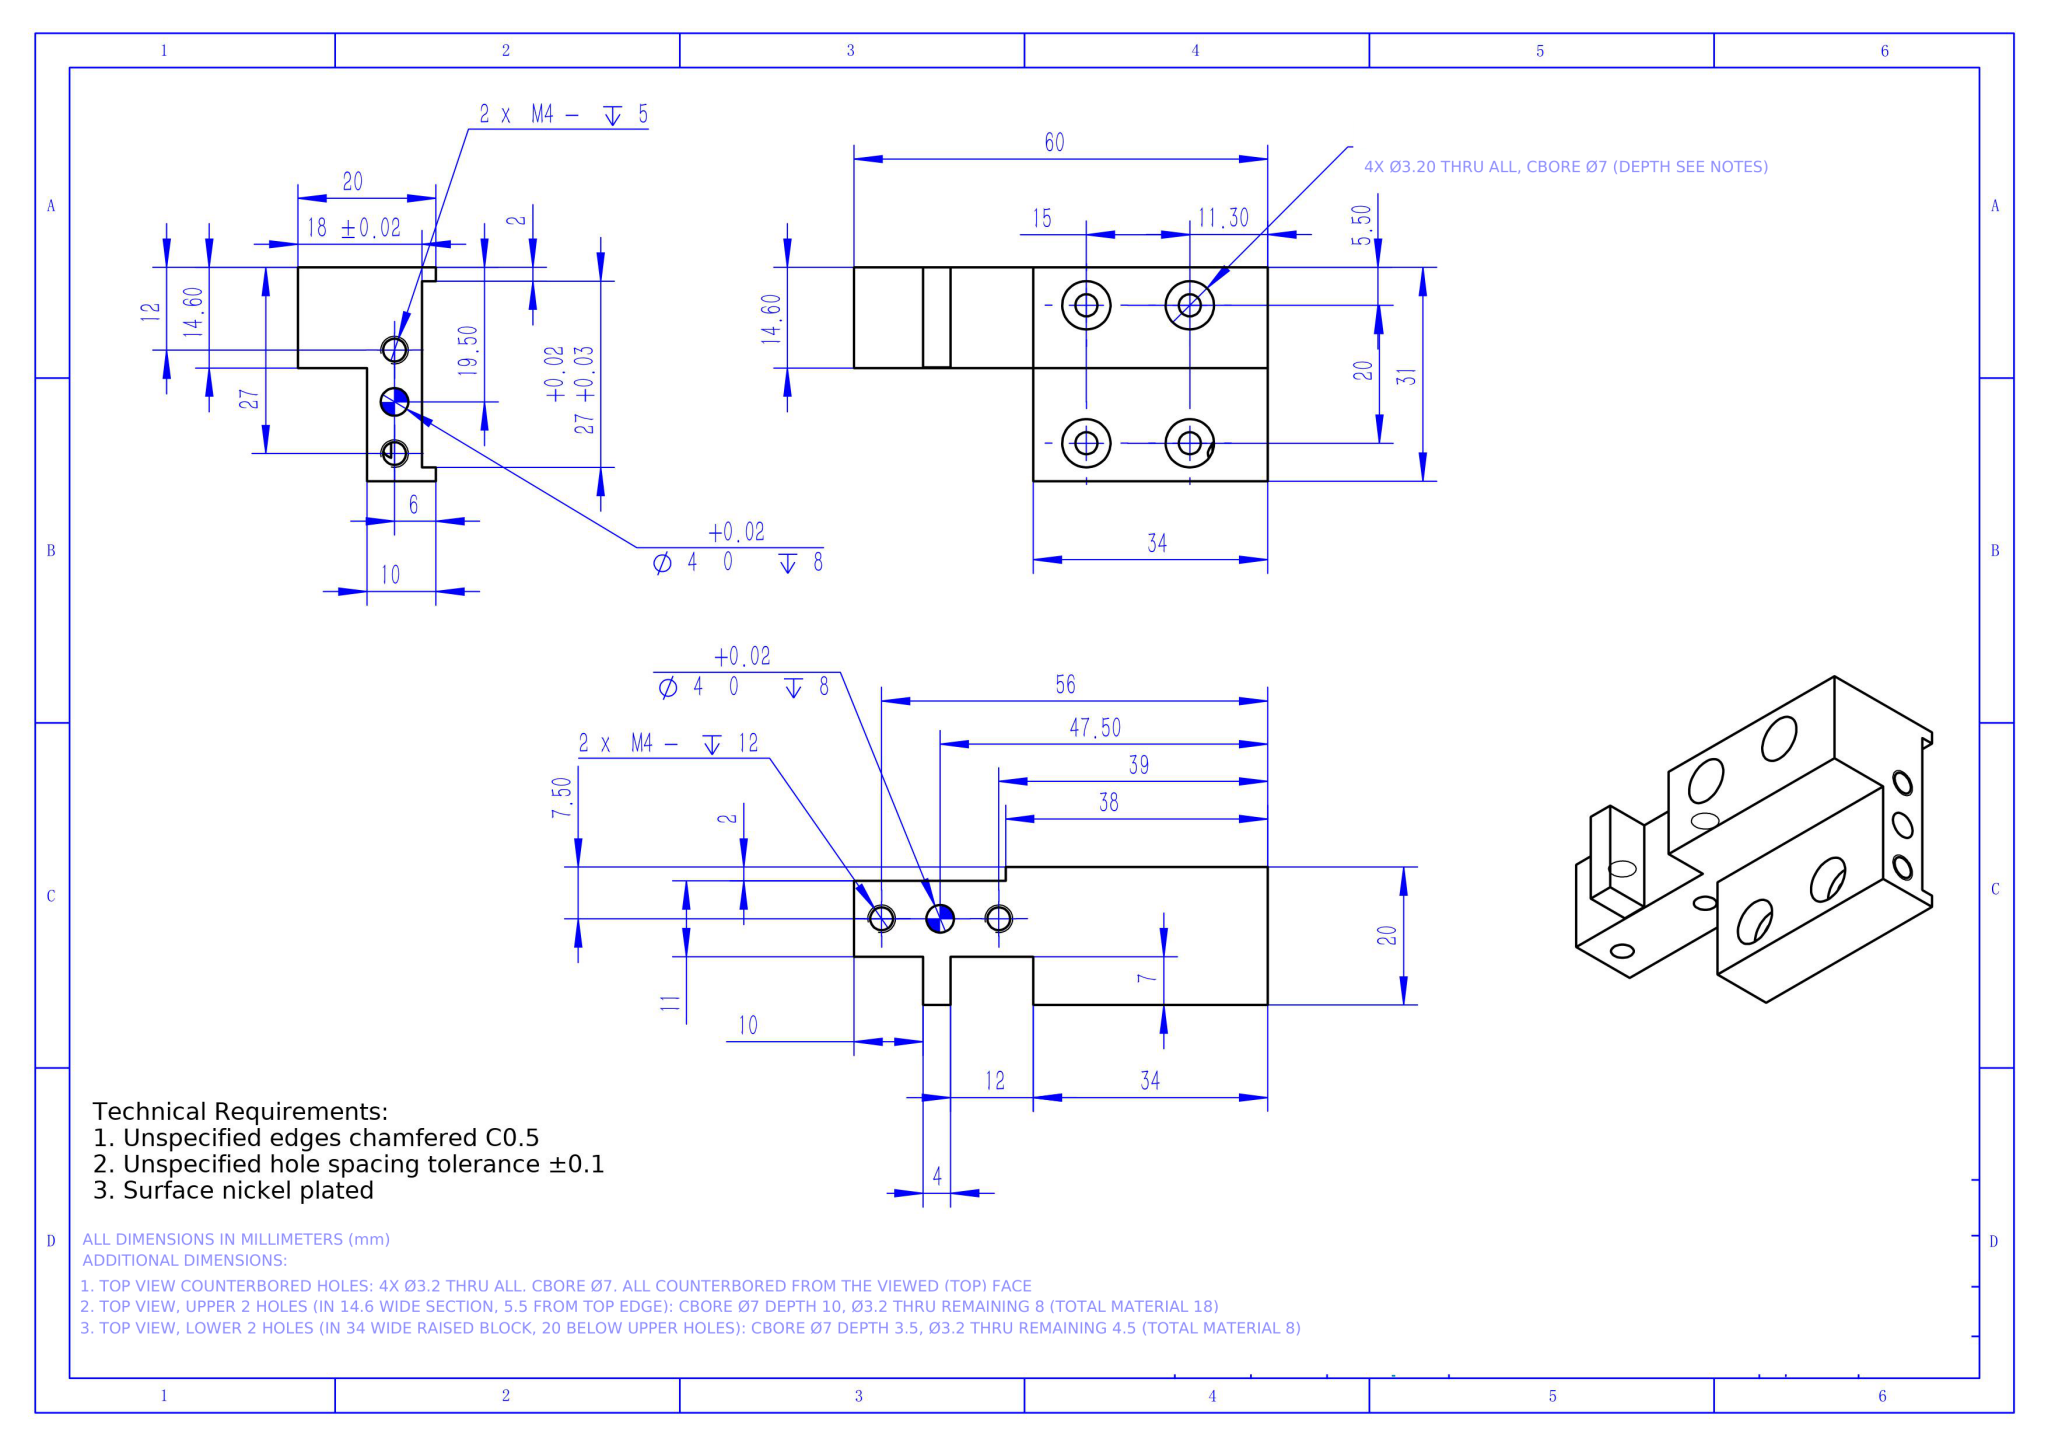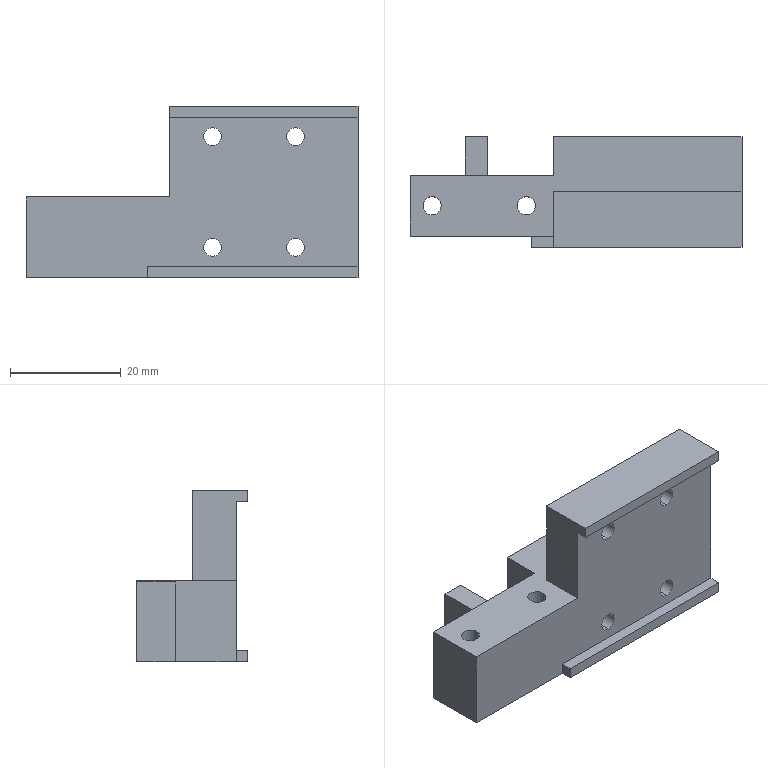Part | NX | mm | 1 solid | 60 faces | box 60 x 20 x 31 mm | volume 16423 mm3 | cylinder 28 | plane 24 | cone 8 | commonest cylinder face diameters 3.3 x8 7 x8 3.2 x8 4 x4